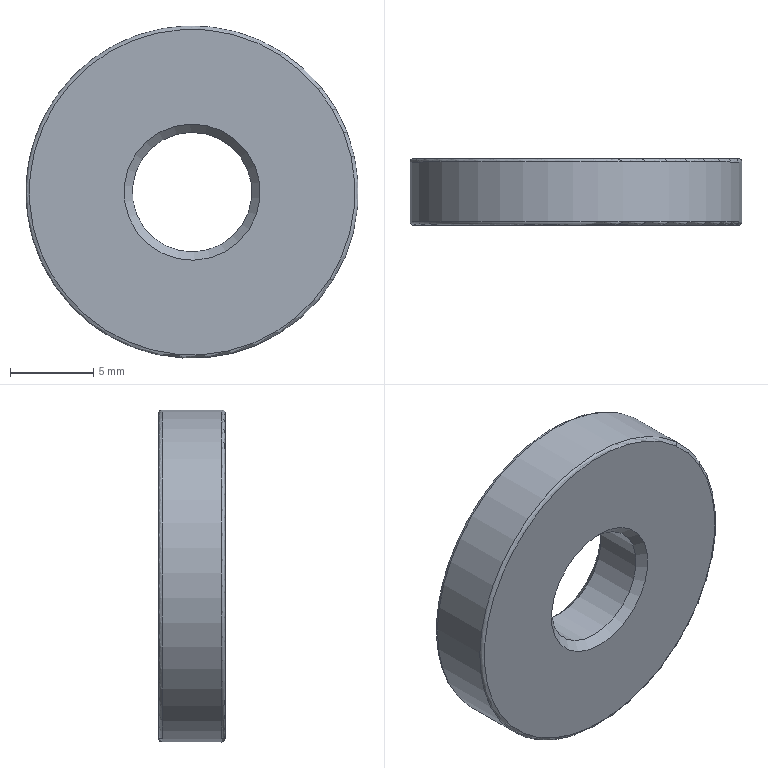Component | NX | TONGTAO | 1 solid | 8 faces | volume 1087 mm3 | cylinder 2 | plane 2 | cone 2 | torus 2 | commonest cylinder face diameters 20 x1 7.2 x1